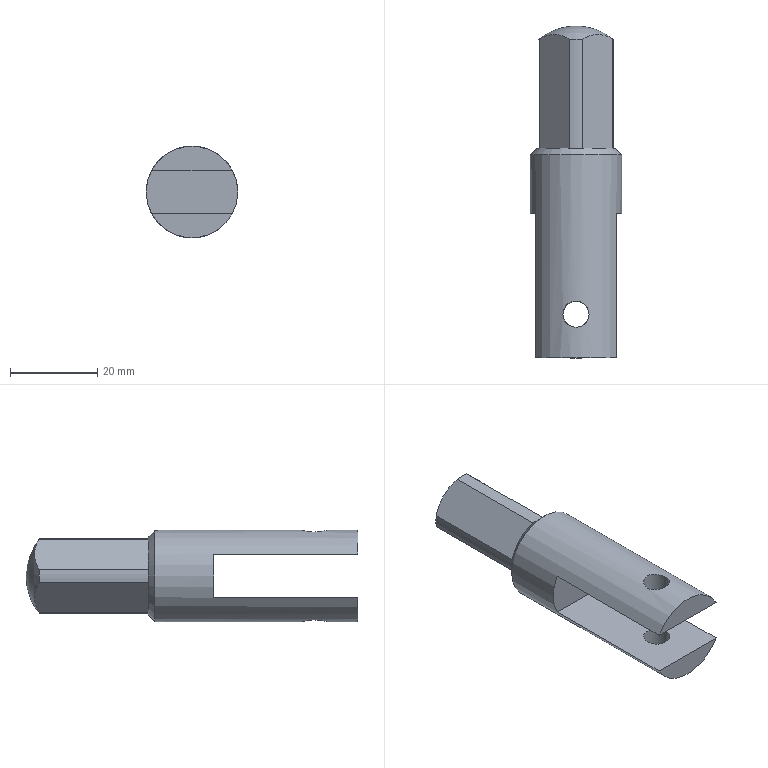Component | NX | SLEEVE_2 | 1 solid | 19 faces | volume 14620 mm3 | plane 10 | cylinder 7 | cone 1 | sphere 1 | commonest cylinder face diameters 17 x4 6 x2 21 x1